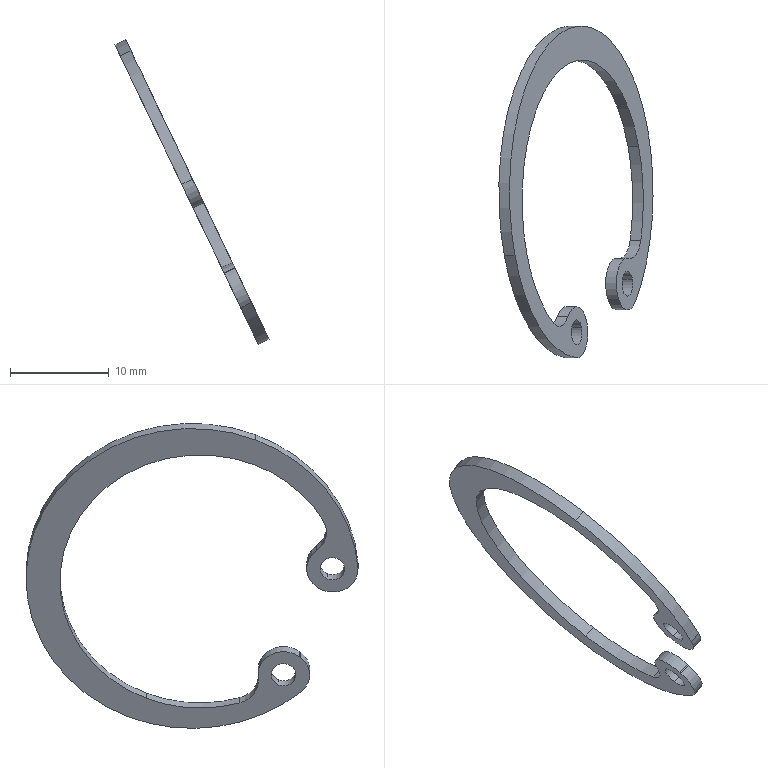Component | SolidWorks | AHTF30S5M100-1_RTWN32-1 | 1 solid | 21 faces | box 15.63 x 33.67 x 30.91 mm | volume 309 mm3 | cylinder 17 | plane 4 | commonest cylinder face diameters 5.2 x5 2.5 x4 28.45 x3 33.7 x3 5 x2
build123d program:
from build123d import *

# Parameters (mm, degrees)
BOSS_EXTRUDE1_DEPTH      = 0.6
BOSS_EXTRUDE1_DEPTH_BACK = 0.6
SKETCH1_R                = 1.25


with BuildPart() as part:
    # Sketch1 → Boss-Extrude1 (new, two sides: drawn at the far end of the back side and taken through both)
    with BuildSketch(Plane(origin=(0, 0, 0), x_dir=(0, 0, -1), z_dir=(1, 0, 0)).offset(-BOSS_EXTRUDE1_DEPTH_BACK)):
        with BuildLine():
            Line((-3.99, -13.556), (-3.956, -13.441))
            ThreePointArc((-3.956, -13.441), (-4.838, -10.667), (-7.741, -10.45))
            ThreePointArc((-7.741, -10.45), (-9.511, -10.749), (-11.053, -9.83))
            ThreePointArc((-11.053, -9.83), (0, 13.35), (11.053, -9.83))
            ThreePointArc((11.053, -9.83), (9.511, -10.749), (7.741, -10.45))
            ThreePointArc((7.741, -10.45), (4.838, -10.667), (3.956, -13.441))
            Line((3.956, -13.441), (3.99, -13.556))
            ThreePointArc((3.99, -13.556), (5.388, -15.141), (7.501, -15.088))
            ThreePointArc((7.501, -15.088), (0, 16.85), (-7.501, -15.088))
            ThreePointArc((-7.501, -15.088), (-5.388, -15.141), (-3.99, -13.556))
        make_face()
        with Locations((6.45, -12.707)):
            Circle(SKETCH1_R, mode=Mode.SUBTRACT)
        with Locations((-6.45, -12.707)):
            Circle(SKETCH1_R, mode=Mode.SUBTRACT)
    extrude(amount=BOSS_EXTRUDE1_DEPTH + BOSS_EXTRUDE1_DEPTH_BACK)


solid = part.part

# Placed as in the assembly
solid = solid.moved(Location((-5.543, 250, 455.725), (-155.302, 23.505, 169.606)))
STEP:
#1=COLOUR_RGB('',0.7922,0.8196,0.9333);
#2=FILL_AREA_STYLE_COLOUR('',#1);
#3=FILL_AREA_STYLE('',(#2));
#4=SURFACE_STYLE_FILL_AREA(#3);
#5=SURFACE_SIDE_STYLE('',(#4));
#6=SURFACE_STYLE_USAGE(.BOTH.,#5);
#7=PRESENTATION_STYLE_ASSIGNMENT((#6));
#8=CARTESIAN_POINT('',(-0.03588,9.497,17.506));
#9=VERTEX_POINT('',#8);
#10=CARTESIAN_POINT('',(-0.07514,9.459,17.588));
#11=VERTEX_POINT('',#10);
#12=CARTESIAN_POINT('',(-0.05551,9.478,17.547));
#13=DIRECTION('',(-0.902,0.,-0.4318));
#14=DIRECTION('',(-0.3988,-0.3832,0.8331));
#15=AXIS2_PLACEMENT_3D('',#12,#13,#14);
#16=CIRCLE('',#15,0.04921);
#17=EDGE_CURVE('',#9,#11,#16,.T.);
#18=ORIENTED_EDGE('',*,*,#17,.T.);
#19=CARTESIAN_POINT('',(-0.03252,9.459,17.609));
#20=VERTEX_POINT('',#19);
#21=CARTESIAN_POINT('',(-0.07514,9.459,17.588));
#22=DIRECTION('',(0.902,-0.,0.4318));
#23=VECTOR('',#22,39.37);
#24=LINE('',#21,#23);
#25=EDGE_CURVE('',#11,#20,#24,.T.);
#26=ORIENTED_EDGE('',*,*,#25,.T.);
#27=CARTESIAN_POINT('',(0.006732,9.497,17.527));
#28=VERTEX_POINT('',#27);
#29=CARTESIAN_POINT('',(-0.0129,9.478,17.568));
#30=DIRECTION('',(-0.902,0.,-0.4318));
#31=DIRECTION('',(-0.3988,-0.3832,0.8331));
#32=AXIS2_PLACEMENT_3D('',#29,#30,#31);
#33=CIRCLE('',#32,0.04921);
#34=EDGE_CURVE('',#28,#20,#33,.T.);
#35=ORIENTED_EDGE('',*,*,#34,.F.);
#36=CARTESIAN_POINT('',(-0.03588,9.497,17.506));
#37=DIRECTION('',(0.902,-0.,0.4318));
#38=VECTOR('',#37,39.37);
#39=LINE('',#36,#38);
#40=EDGE_CURVE('',#9,#28,#39,.T.);
#41=ORIENTED_EDGE('',*,*,#40,.F.);
#42=EDGE_LOOP('',(#18,#26,#35,#41));
#43=FACE_OUTER_BOUND('',#42,.T.);
#44=CARTESIAN_POINT('',(-0.05551,9.478,17.547));
#45=DIRECTION('',(0.902,-0.,0.4318));
#46=DIRECTION('',(0.3988,0.3832,-0.8331));
#47=AXIS2_PLACEMENT_3D('',#44,#45,#46);
#48=CYLINDRICAL_SURFACE('',#47,0.04921);
#49=ADVANCED_FACE('',(#43),#48,.F.);
#50=CARTESIAN_POINT('',(-0.2384,9.302,17.929));
#51=VERTEX_POINT('',#50);
#52=CARTESIAN_POINT('',(-0.2777,9.264,18.011));
#53=VERTEX_POINT('',#52);
#54=CARTESIAN_POINT('',(-0.2581,9.283,17.97));
#55=DIRECTION('',(-0.902,0.,-0.4318));
#56=DIRECTION('',(-0.3988,-0.3832,0.8331));
#57=AXIS2_PLACEMENT_3D('',#54,#55,#56);
#58=CIRCLE('',#57,0.04921);
#59=EDGE_CURVE('',#51,#53,#58,.T.);
#60=ORIENTED_EDGE('',*,*,#59,.T.);
#61=CARTESIAN_POINT('',(-0.2351,9.264,18.032));
#62=VERTEX_POINT('',#61);
#63=CARTESIAN_POINT('',(-0.2777,9.264,18.011));
#64=DIRECTION('',(0.902,-0.,0.4318));
#65=VECTOR('',#64,39.37);
#66=LINE('',#63,#65);
#67=EDGE_CURVE('',#53,#62,#66,.T.);
#68=ORIENTED_EDGE('',*,*,#67,.T.);
#69=CARTESIAN_POINT('',(-0.1958,9.302,17.95));
#70=VERTEX_POINT('',#69);
#71=CARTESIAN_POINT('',(-0.2155,9.283,17.991));
#72=DIRECTION('',(-0.902,0.,-0.4318));
#73=DIRECTION('',(-0.3988,-0.3832,0.8331));
#74=AXIS2_PLACEMENT_3D('',#71,#72,#73);
#75=CIRCLE('',#74,0.04921);
#76=EDGE_CURVE('',#70,#62,#75,.T.);
#77=ORIENTED_EDGE('',*,*,#76,.F.);
#78=CARTESIAN_POINT('',(-0.2384,9.302,17.929));
#79=DIRECTION('',(0.902,-0.,0.4318));
#80=VECTOR('',#79,39.37);
#81=LINE('',#78,#80);
#82=EDGE_CURVE('',#51,#70,#81,.T.);
#83=ORIENTED_EDGE('',*,*,#82,.F.);
#84=EDGE_LOOP('',(#60,#68,#77,#83));
#85=FACE_OUTER_BOUND('',#84,.T.);
#86=CARTESIAN_POINT('',(-0.2581,9.283,17.97));
#87=DIRECTION('',(0.902,-0.,0.4318));
#88=DIRECTION('',(0.3988,0.3832,-0.8331));
#89=AXIS2_PLACEMENT_3D('',#86,#87,#88);
#90=CYLINDRICAL_SURFACE('',#89,0.04921);
#91=ADVANCED_FACE('',(#85),#90,.F.);
#92=CARTESIAN_POINT('',(-0.2172,9.322,17.885));
#93=VERTEX_POINT('',#92);
#94=CARTESIAN_POINT('',(-0.2141,9.294,17.879));
#95=VERTEX_POINT('',#94);
#96=CARTESIAN_POINT('',(-0.2581,9.283,17.97));
#97=DIRECTION('',(-0.902,0.,-0.4318));
#98=DIRECTION('',(-0.3988,-0.3832,0.8331));
#99=AXIS2_PLACEMENT_3D('',#96,#97,#98);
#100=CIRCLE('',#99,0.1024);
#101=EDGE_CURVE('',#93,#95,#100,.T.);
#102=ORIENTED_EDGE('',*,*,#101,.F.);
#103=CARTESIAN_POINT('',(-0.1746,9.322,17.906));
#104=VERTEX_POINT('',#103);
#105=CARTESIAN_POINT('',(-0.2172,9.322,17.885));
#106=DIRECTION('',(0.902,-0.,0.4318));
#107=VECTOR('',#106,39.37);
#108=LINE('',#105,#107);
#109=EDGE_CURVE('',#93,#104,#108,.T.);
#110=ORIENTED_EDGE('',*,*,#109,.T.);
#111=CARTESIAN_POINT('',(-0.1715,9.294,17.899));
#112=VERTEX_POINT('',#111);
#113=CARTESIAN_POINT('',(-0.2155,9.283,17.991));
#114=DIRECTION('',(-0.902,0.,-0.4318));
#115=DIRECTION('',(-0.3988,-0.3832,0.8331));
#116=AXIS2_PLACEMENT_3D('',#113,#114,#115);
#117=CIRCLE('',#116,0.1024);
#118=EDGE_CURVE('',#104,#112,#117,.T.);
#119=ORIENTED_EDGE('',*,*,#118,.T.);
#120=CARTESIAN_POINT('',(-0.2141,9.294,17.879));
#121=DIRECTION('',(0.902,-0.,0.4318));
#122=VECTOR('',#121,39.37);
#123=LINE('',#120,#122);
#124=EDGE_CURVE('',#95,#112,#123,.T.);
#125=ORIENTED_EDGE('',*,*,#124,.F.);
#126=EDGE_LOOP('',(#102,#110,#119,#125));
#127=FACE_OUTER_BOUND('',#126,.T.);
#128=CARTESIAN_POINT('',(-0.2581,9.283,17.97));
#129=DIRECTION('',(0.902,-0.,0.4318));
#130=DIRECTION('',(0.3988,0.3832,-0.8331));
#131=AXIS2_PLACEMENT_3D('',#128,#129,#130);
#132=CYLINDRICAL_SURFACE('',#131,0.1024);
#133=ADVANCED_FACE('',(#127),#132,.T.);
#134=CARTESIAN_POINT('',(-0.4572,9.596,18.386));
#135=VERTEX_POINT('',#134);
#136=CARTESIAN_POINT('',(-0.3491,9.318,18.161));
#137=VERTEX_POINT('',#136);
#138=CARTESIAN_POINT('',(-0.2339,9.811,17.92));
#139=DIRECTION('',(0.902,-0.,0.4318));
#140=DIRECTION('',(0.3988,0.3832,-0.8331));
#141=AXIS2_PLACEMENT_3D('',#138,#139,#140);
#142=CIRCLE('',#141,0.56);
#143=EDGE_CURVE('',#135,#137,#142,.T.);
#144=ORIENTED_EDGE('',*,*,#143,.F.);
#145=CARTESIAN_POINT('',(-0.4146,9.596,18.407));
#146=VERTEX_POINT('',#145);
#147=CARTESIAN_POINT('',(-0.4572,9.596,18.386));
#148=DIRECTION('',(0.902,-0.,0.4318));
#149=VECTOR('',#148,39.37);
#150=LINE('',#147,#149);
#151=EDGE_CURVE('',#135,#146,#150,.T.);
#152=ORIENTED_EDGE('',*,*,#151,.T.);
#153=CARTESIAN_POINT('',(-0.3065,9.318,18.181));
#154=VERTEX_POINT('',#153);
#155=CARTESIAN_POINT('',(-0.1912,9.811,17.94));
#156=DIRECTION('',(0.902,-0.,0.4318));
#157=DIRECTION('',(0.3988,0.3832,-0.8331));
#158=AXIS2_PLACEMENT_3D('',#155,#156,#157);
#159=CIRCLE('',#158,0.56);
#160=EDGE_CURVE('',#146,#154,#159,.T.);
#161=ORIENTED_EDGE('',*,*,#160,.T.);
#162=CARTESIAN_POINT('',(-0.3491,9.318,18.161));
#163=DIRECTION('',(0.902,-0.,0.4318));
#164=VECTOR('',#163,39.37);
#165=LINE('',#162,#164);
#166=EDGE_CURVE('',#137,#154,#165,.T.);
#167=ORIENTED_EDGE('',*,*,#166,.F.);
#168=EDGE_LOOP('',(#144,#152,#161,#167));
#169=FACE_OUTER_BOUND('',#168,.T.);
#170=CARTESIAN_POINT('',(-0.2339,9.811,17.92));
#171=DIRECTION('',(0.902,-0.,0.4318));
#172=DIRECTION('',(0.3988,0.3832,-0.8331));
#173=AXIS2_PLACEMENT_3D('',#170,#171,#172);
#174=CYLINDRICAL_SURFACE('',#173,0.56);
#175=ADVANCED_FACE('',(#169),#174,.F.);
#176=ORIENTED_EDGE('',*,*,#151,.F.);
#177=CARTESIAN_POINT('',(-0.01049,10.025,17.453));
#178=VERTEX_POINT('',#177);
#179=CARTESIAN_POINT('',(-0.2339,9.811,17.92));
#180=DIRECTION('',(0.902,-0.,0.4318));
#181=DIRECTION('',(0.3988,0.3832,-0.8331));
#182=AXIS2_PLACEMENT_3D('',#179,#180,#181);
#183=CIRCLE('',#182,0.56);
#184=EDGE_CURVE('',#178,#135,#183,.T.);
#185=ORIENTED_EDGE('',*,*,#184,.F.);
#186=CARTESIAN_POINT('',(0.03212,10.025,17.474));
#187=VERTEX_POINT('',#186);
#188=CARTESIAN_POINT('',(-0.01049,10.025,17.453));
#189=DIRECTION('',(0.902,-0.,0.4318));
#190=VECTOR('',#189,39.37);
#191=LINE('',#188,#190);
#192=EDGE_CURVE('',#178,#187,#191,.T.);
#193=ORIENTED_EDGE('',*,*,#192,.T.);
#194=CARTESIAN_POINT('',(-0.1912,9.811,17.94));
#195=DIRECTION('',(0.902,-0.,0.4318));
#196=DIRECTION('',(0.3988,0.3832,-0.8331));
#197=AXIS2_PLACEMENT_3D('',#194,#195,#196);
#198=CIRCLE('',#197,0.56);
#199=EDGE_CURVE('',#187,#146,#198,.T.);
#200=ORIENTED_EDGE('',*,*,#199,.T.);
#201=EDGE_LOOP('',(#176,#185,#193,#200));
#202=FACE_OUTER_BOUND('',#201,.T.);
#203=CARTESIAN_POINT('',(-0.2339,9.811,17.92));
#204=DIRECTION('',(0.902,-0.,0.4318));
#205=DIRECTION('',(0.3988,0.3832,-0.8331));
#206=AXIS2_PLACEMENT_3D('',#203,#204,#205);
#207=CYLINDRICAL_SURFACE('',#206,0.56);
#208=ADVANCED_FACE('',(#202),#207,.F.);
#209=CARTESIAN_POINT('',(-0.5041,9.588,18.484));
#210=VERTEX_POINT('',#209);
#211=CARTESIAN_POINT('',(0.02503,10.097,17.379));
#212=VERTEX_POINT('',#211);
#213=CARTESIAN_POINT('',(-0.2396,9.843,17.932));
#214=DIRECTION('',(-0.902,0.,-0.4318));
#215=DIRECTION('',(-0.3988,-0.3832,0.8331));
#216=AXIS2_PLACEMENT_3D('',#213,#214,#215);
#217=CIRCLE('',#216,0.6634);
#218=EDGE_CURVE('',#210,#212,#217,.T.);
#219=ORIENTED_EDGE('',*,*,#218,.F.);
#220=CARTESIAN_POINT('',(-0.4615,9.588,18.505));
#221=VERTEX_POINT('',#220);
#222=CARTESIAN_POINT('',(-0.5041,9.588,18.484));
#223=DIRECTION('',(0.902,-0.,0.4318));
#224=VECTOR('',#223,39.37);
#225=LINE('',#222,#224);
#226=EDGE_CURVE('',#210,#221,#225,.T.);
#227=ORIENTED_EDGE('',*,*,#226,.T.);
#228=CARTESIAN_POINT('',(0.06764,10.097,17.399));
#229=VERTEX_POINT('',#228);
#230=CARTESIAN_POINT('',(-0.1969,9.843,17.952));
#231=DIRECTION('',(-0.902,0.,-0.4318));
#232=DIRECTION('',(-0.3988,-0.3832,0.8331));
#233=AXIS2_PLACEMENT_3D('',#230,#231,#232);
#234=CIRCLE('',#233,0.6634);
#235=EDGE_CURVE('',#221,#229,#234,.T.);
#236=ORIENTED_EDGE('',*,*,#235,.T.);
#237=CARTESIAN_POINT('',(0.02503,10.097,17.379));
#238=DIRECTION('',(0.902,-0.,0.4318));
#239=VECTOR('',#238,39.37);
#240=LINE('',#237,#239);
#241=EDGE_CURVE('',#212,#229,#240,.T.);
#242=ORIENTED_EDGE('',*,*,#241,.F.);
#243=EDGE_LOOP('',(#219,#227,#236,#242));
#244=FACE_OUTER_BOUND('',#243,.T.);
#245=CARTESIAN_POINT('',(-0.2396,9.843,17.932));
#246=DIRECTION('',(0.902,-0.,0.4318));
#247=DIRECTION('',(0.3988,0.3832,-0.8331));
#248=AXIS2_PLACEMENT_3D('',#245,#246,#247);
#249=CYLINDRICAL_SURFACE('',#248,0.6634);
#250=ADVANCED_FACE('',(#244),#249,.T.);
#251=CARTESIAN_POINT('',(-0.0235,9.407,17.48));
#252=VERTEX_POINT('',#251);
#253=CARTESIAN_POINT('',(-0.2396,9.843,17.932));
#254=DIRECTION('',(-0.902,0.,-0.4318));
#255=DIRECTION('',(-0.3988,-0.3832,0.8331));
#256=AXIS2_PLACEMENT_3D('',#253,#254,#255);
#257=CIRCLE('',#256,0.6634);
#258=EDGE_CURVE('',#212,#252,#257,.T.);
#259=ORIENTED_EDGE('',*,*,#258,.F.);
#260=ORIENTED_EDGE('',*,*,#241,.T.);
#261=CARTESIAN_POINT('',(0.01912,9.407,17.501));
#262=VERTEX_POINT('',#261);
#263=CARTESIAN_POINT('',(-0.1969,9.843,17.952));
#264=DIRECTION('',(-0.902,0.,-0.4318));
#265=DIRECTION('',(-0.3988,-0.3832,0.8331));
#266=AXIS2_PLACEMENT_3D('',#263,#264,#265);
#267=CIRCLE('',#266,0.6634);
#268=EDGE_CURVE('',#229,#262,#267,.T.);
#269=ORIENTED_EDGE('',*,*,#268,.T.);
#270=CARTESIAN_POINT('',(-0.0235,9.407,17.48));
#271=DIRECTION('',(0.902,-0.,0.4318));
#272=VECTOR('',#271,39.37);
#273=LINE('',#270,#272);
#274=EDGE_CURVE('',#252,#262,#273,.T.);
#275=ORIENTED_EDGE('',*,*,#274,.F.);
#276=EDGE_LOOP('',(#259,#260,#269,#275));
#277=FACE_OUTER_BOUND('',#276,.T.);
#278=CARTESIAN_POINT('',(-0.2396,9.843,17.932));
#279=DIRECTION('',(0.902,-0.,0.4318));
#280=DIRECTION('',(0.3988,0.3832,-0.8331));
#281=AXIS2_PLACEMENT_3D('',#278,#279,#280);
#282=CYLINDRICAL_SURFACE('',#281,0.6634);
#283=ADVANCED_FACE('',(#277),#282,.T.);
#284=ORIENTED_EDGE('',*,*,#59,.F.);
#285=CARTESIAN_POINT('',(-0.2581,9.283,17.97));
#286=DIRECTION('',(-0.902,0.,-0.4318));
#287=DIRECTION('',(-0.3988,-0.3832,0.8331));
#288=AXIS2_PLACEMENT_3D('',#285,#286,#287);
#289=CIRCLE('',#288,0.04921);
#290=EDGE_CURVE('',#53,#51,#289,.T.);
#291=ORIENTED_EDGE('',*,*,#290,.F.);
#292=EDGE_LOOP('',(#284,#291));
#293=FACE_BOUND('',#292,.T.);
#294=CARTESIAN_POINT('',(-0.2139,9.289,17.878));
#295=VERTEX_POINT('',#294);
#296=CARTESIAN_POINT('',(-0.259,9.181,17.972));
#297=VERTEX_POINT('',#296);
#298=CARTESIAN_POINT('',(-0.2562,9.279,17.966));
#299=DIRECTION('',(-0.902,0.,-0.4318));
#300=DIRECTION('',(-0.3988,-0.3832,0.8331));
#301=AXIS2_PLACEMENT_3D('',#298,#299,#300);
#302=CIRCLE('',#301,0.09843);
#303=EDGE_CURVE('',#295,#297,#302,.T.);
#304=ORIENTED_EDGE('',*,*,#303,.T.);
#305=CARTESIAN_POINT('',(-0.2396,9.843,17.932));
#306=DIRECTION('',(-0.902,0.,-0.4318));
#307=DIRECTION('',(-0.3988,-0.3832,0.8331));
#308=AXIS2_PLACEMENT_3D('',#305,#306,#307);
#309=CIRCLE('',#308,0.6634);
#310=EDGE_CURVE('',#297,#210,#309,.T.);
#311=ORIENTED_EDGE('',*,*,#310,.T.);
#312=ORIENTED_EDGE('',*,*,#218,.T.);
#313=ORIENTED_EDGE('',*,*,#258,.T.);
#314=CARTESIAN_POINT('',(-0.08861,9.41,17.616));
#315=VERTEX_POINT('',#314);
#316=CARTESIAN_POINT('',(-0.05555,9.472,17.547));
#317=DIRECTION('',(-0.902,0.,-0.4318));
#318=DIRECTION('',(-0.3988,-0.3832,0.8331));
#319=AXIS2_PLACEMENT_3D('',#316,#317,#318);
#320=CIRCLE('',#319,0.09843);
#321=EDGE_CURVE('',#252,#315,#320,.T.);
#322=ORIENTED_EDGE('',*,*,#321,.T.);
#323=CARTESIAN_POINT('',(-0.08989,9.413,17.619));
#324=VERTEX_POINT('',#323);
#325=CARTESIAN_POINT('',(-0.08861,9.41,17.616));
#326=DIRECTION('',(-0.2713,0.7779,0.5668));
#327=VECTOR('',#326,39.37);
#328=LINE('',#325,#327);
#329=EDGE_CURVE('',#315,#324,#328,.T.);
#330=ORIENTED_EDGE('',*,*,#329,.T.);
#331=CARTESIAN_POINT('',(-0.04993,9.579,17.536));
#332=VERTEX_POINT('',#331);
#333=CARTESIAN_POINT('',(-0.05551,9.478,17.547));
#334=DIRECTION('',(-0.902,0.,-0.4318));
#335=DIRECTION('',(-0.3988,-0.3832,0.8331));
#336=AXIS2_PLACEMENT_3D('',#333,#334,#335);
#337=CIRCLE('',#336,0.1024);
#338=EDGE_CURVE('',#324,#332,#337,.T.);
#339=ORIENTED_EDGE('',*,*,#338,.T.);
#340=CARTESIAN_POINT('',(-0.001977,9.652,17.435));
#341=VERTEX_POINT('',#340);
#342=CARTESIAN_POINT('',(-0.04436,9.681,17.524));
#343=DIRECTION('',(0.902,-0.,0.4318));
#344=DIRECTION('',(0.3988,0.3832,-0.8331));
#345=AXIS2_PLACEMENT_3D('',#342,#343,#344);
#346=CIRCLE('',#345,0.1024);
#347=EDGE_CURVE('',#332,#341,#346,.T.);
#348=ORIENTED_EDGE('',*,*,#347,.T.);
#349=CARTESIAN_POINT('',(-0.2339,9.811,17.92));
#350=DIRECTION('',(0.902,-0.,0.4318));
#351=DIRECTION('',(0.3988,0.3832,-0.8331));
#352=AXIS2_PLACEMENT_3D('',#349,#350,#351);
#353=CIRCLE('',#352,0.56);
#354=EDGE_CURVE('',#341,#178,#353,.T.);
#355=ORIENTED_EDGE('',*,*,#354,.T.);
#356=ORIENTED_EDGE('',*,*,#184,.T.);
#357=ORIENTED_EDGE('',*,*,#143,.T.);
#358=CARTESIAN_POINT('',(-0.293,9.346,18.043));
#359=VERTEX_POINT('',#358);
#360=CARTESIAN_POINT('',(-0.328,9.408,18.117));
#361=DIRECTION('',(0.902,-0.,0.4318));
#362=DIRECTION('',(0.3988,0.3832,-0.8331));
#363=AXIS2_PLACEMENT_3D('',#360,#361,#362);
#364=CIRCLE('',#363,0.1024);
#365=EDGE_CURVE('',#137,#359,#364,.T.);
#366=ORIENTED_EDGE('',*,*,#365,.T.);
#367=CARTESIAN_POINT('',(-0.2581,9.283,17.97));
#368=DIRECTION('',(-0.902,0.,-0.4318));
#369=DIRECTION('',(-0.3988,-0.3832,0.8331));
#370=AXIS2_PLACEMENT_3D('',#367,#368,#369);
#371=CIRCLE('',#370,0.1024);
#372=EDGE_CURVE('',#359,#93,#371,.T.);
#373=ORIENTED_EDGE('',*,*,#372,.T.);
#374=ORIENTED_EDGE('',*,*,#101,.T.);
#375=CARTESIAN_POINT('',(-0.2141,9.294,17.879));
#376=DIRECTION('',(0.04611,-0.9943,-0.09632));
#377=VECTOR('',#376,39.37);
#378=LINE('',#375,#377);
#379=EDGE_CURVE('',#95,#295,#378,.T.);
#380=ORIENTED_EDGE('',*,*,#379,.T.);
#381=EDGE_LOOP('',(#304,#311,#312,#313,#322,#330,#339,#348,#355,#356,#357,#366,#373,#374,#380));
#382=FACE_OUTER_BOUND('',#381,.T.);
#383=ORIENTED_EDGE('',*,*,#17,.F.);
#384=CARTESIAN_POINT('',(-0.05551,9.478,17.547));
#385=DIRECTION('',(-0.902,0.,-0.4318));
#386=DIRECTION('',(-0.3988,-0.3832,0.8331));
#387=AXIS2_PLACEMENT_3D('',#384,#385,#386);
#388=CIRCLE('',#387,0.04921);
#389=EDGE_CURVE('',#11,#9,#388,.T.);
#390=ORIENTED_EDGE('',*,*,#389,.F.);
#391=EDGE_LOOP('',(#383,#390));
#392=FACE_BOUND('',#391,.T.);
#393=CARTESIAN_POINT('',(-0.2562,9.279,17.966));
#394=DIRECTION('',(-0.902,0.,-0.4318));
#395=DIRECTION('',(-0.3988,-0.3832,0.8331));
#396=AXIS2_PLACEMENT_3D('',#393,#394,#395);
#397=PLANE('',#396);
#398=ADVANCED_FACE('',(#293,#382,#392),#397,.T.);
#399=CARTESIAN_POINT('',(-0.1713,9.289,17.899));
#400=VERTEX_POINT('',#399);
#401=CARTESIAN_POINT('',(-0.2139,9.289,17.878));
#402=DIRECTION('',(0.902,-0.,0.4318));
#403=VECTOR('',#402,39.37);
#404=LINE('',#401,#403);
#405=EDGE_CURVE('',#295,#400,#404,.T.);
#406=ORIENTED_EDGE('',*,*,#405,.T.);
#407=CARTESIAN_POINT('',(-0.2164,9.181,17.993));
#408=VERTEX_POINT('',#407);
#409=CARTESIAN_POINT('',(-0.2135,9.279,17.987));
#410=DIRECTION('',(-0.902,0.,-0.4318));
#411=DIRECTION('',(-0.3988,-0.3832,0.8331));
#412=AXIS2_PLACEMENT_3D('',#409,#410,#411);
#413=CIRCLE('',#412,0.09843);
#414=EDGE_CURVE('',#400,#408,#413,.T.);
#415=ORIENTED_EDGE('',*,*,#414,.T.);
#416=CARTESIAN_POINT('',(-0.259,9.181,17.972));
#417=DIRECTION('',(0.902,-0.,0.4318));
#418=VECTOR('',#417,39.37);
#419=LINE('',#416,#418);
#420=EDGE_CURVE('',#297,#408,#419,.T.);
#421=ORIENTED_EDGE('',*,*,#420,.F.);
#422=ORIENTED_EDGE('',*,*,#303,.F.);
#423=EDGE_LOOP('',(#406,#415,#421,#422));
#424=FACE_OUTER_BOUND('',#423,.T.);
#425=CARTESIAN_POINT('',(-0.2562,9.279,17.966));
#426=DIRECTION('',(0.902,-0.,0.4318));
#427=DIRECTION('',(0.3988,0.3832,-0.8331));
#428=AXIS2_PLACEMENT_3D('',#425,#426,#427);
#429=CYLINDRICAL_SURFACE('',#428,0.09843);
#430=ADVANCED_FACE('',(#424),#429,.T.);
#431=ORIENTED_EDGE('',*,*,#226,.F.);
#432=ORIENTED_EDGE('',*,*,#310,.F.);
#433=ORIENTED_EDGE('',*,*,#420,.T.);
#434=CARTESIAN_POINT('',(-0.1969,9.843,17.952));
#435=DIRECTION('',(-0.902,0.,-0.4318));
#436=DIRECTION('',(-0.3988,-0.3832,0.8331));
#437=AXIS2_PLACEMENT_3D('',#434,#435,#436);
#438=CIRCLE('',#437,0.6634);
#439=EDGE_CURVE('',#408,#221,#438,.T.);
#440=ORIENTED_EDGE('',*,*,#439,.T.);
#441=EDGE_LOOP('',(#431,#432,#433,#440));
#442=FACE_OUTER_BOUND('',#441,.T.);
#443=CARTESIAN_POINT('',(-0.2396,9.843,17.932));
#444=DIRECTION('',(0.902,-0.,0.4318));
#445=DIRECTION('',(0.3988,0.3832,-0.8331));
#446=AXIS2_PLACEMENT_3D('',#443,#444,#445);
#447=CYLINDRICAL_SURFACE('',#446,0.6634);
#448=ADVANCED_FACE('',(#442),#447,.T.);
#449=ORIENTED_EDGE('',*,*,#274,.T.);
#450=CARTESIAN_POINT('',(-0.046,9.41,17.637));
#451=VERTEX_POINT('',#450);
#452=CARTESIAN_POINT('',(-0.01294,9.472,17.568));
#453=DIRECTION('',(-0.902,0.,-0.4318));
#454=DIRECTION('',(-0.3988,-0.3832,0.8331));
#455=AXIS2_PLACEMENT_3D('',#452,#453,#454);
#456=CIRCLE('',#455,0.09843);
#457=EDGE_CURVE('',#262,#451,#456,.T.);
#458=ORIENTED_EDGE('',*,*,#457,.T.);
#459=CARTESIAN_POINT('',(-0.08861,9.41,17.616));
#460=DIRECTION('',(0.902,-0.,0.4318));
#461=VECTOR('',#460,39.37);
#462=LINE('',#459,#461);
#463=EDGE_CURVE('',#315,#451,#462,.T.);
#464=ORIENTED_EDGE('',*,*,#463,.F.);
#465=ORIENTED_EDGE('',*,*,#321,.F.);
#466=EDGE_LOOP('',(#449,#458,#464,#465));
#467=FACE_OUTER_BOUND('',#466,.T.);
#468=CARTESIAN_POINT('',(-0.05555,9.472,17.547));
#469=DIRECTION('',(0.902,-0.,0.4318));
#470=DIRECTION('',(0.3988,0.3832,-0.8331));
#471=AXIS2_PLACEMENT_3D('',#468,#469,#470);
#472=CYLINDRICAL_SURFACE('',#471,0.09843);
#473=ADVANCED_FACE('',(#467),#472,.T.);
#474=ORIENTED_EDGE('',*,*,#463,.T.);
#475=CARTESIAN_POINT('',(-0.04728,9.413,17.639));
#476=VERTEX_POINT('',#475);
#477=CARTESIAN_POINT('',(-0.046,9.41,17.637));
#478=DIRECTION('',(-0.2713,0.7779,0.5668));
#479=VECTOR('',#478,39.37);
#480=LINE('',#477,#479);
#481=EDGE_CURVE('',#451,#476,#480,.T.);
#482=ORIENTED_EDGE('',*,*,#481,.T.);
#483=CARTESIAN_POINT('',(-0.08989,9.413,17.619));
#484=DIRECTION('',(0.902,-0.,0.4318));
#485=VECTOR('',#484,39.37);
#486=LINE('',#483,#485);
#487=EDGE_CURVE('',#324,#476,#486,.T.);
#488=ORIENTED_EDGE('',*,*,#487,.F.);
#489=ORIENTED_EDGE('',*,*,#329,.F.);
#490=EDGE_LOOP('',(#474,#482,#488,#489));
#491=FACE_OUTER_BOUND('',#490,.T.);
#492=CARTESIAN_POINT('',(-0.08861,9.41,17.616));
#493=DIRECTION('',(0.3359,0.6284,-0.7017));
#494=DIRECTION('',(0.2713,-0.7779,-0.5668));
#495=AXIS2_PLACEMENT_3D('',#492,#493,#494);
#496=PLANE('',#495);
#497=ADVANCED_FACE('',(#491),#496,.F.);
#498=ORIENTED_EDGE('',*,*,#487,.T.);
#499=CARTESIAN_POINT('',(-0.00732,9.579,17.556));
#500=VERTEX_POINT('',#499);
#501=CARTESIAN_POINT('',(-0.0129,9.478,17.568));
#502=DIRECTION('',(-0.902,0.,-0.4318));
#503=DIRECTION('',(-0.3988,-0.3832,0.8331));
#504=AXIS2_PLACEMENT_3D('',#501,#502,#503);
#505=CIRCLE('',#504,0.1024);
#506=EDGE_CURVE('',#476,#500,#505,.T.);
#507=ORIENTED_EDGE('',*,*,#506,.T.);
#508=CARTESIAN_POINT('',(-0.04993,9.579,17.536));
#509=DIRECTION('',(0.902,-0.,0.4318));
#510=VECTOR('',#509,39.37);
#511=LINE('',#508,#510);
#512=EDGE_CURVE('',#332,#500,#511,.T.);
#513=ORIENTED_EDGE('',*,*,#512,.F.);
#514=ORIENTED_EDGE('',*,*,#338,.F.);
#515=EDGE_LOOP('',(#498,#507,#513,#514));
#516=FACE_OUTER_BOUND('',#515,.T.);
#517=CARTESIAN_POINT('',(-0.05551,9.478,17.547));
#518=DIRECTION('',(0.902,-0.,0.4318));
#519=DIRECTION('',(0.3988,0.3832,-0.8331));
#520=AXIS2_PLACEMENT_3D('',#517,#518,#519);
#521=CYLINDRICAL_SURFACE('',#520,0.1024);
#522=ADVANCED_FACE('',(#516),#521,.T.);
#523=ORIENTED_EDGE('',*,*,#512,.T.);
#524=CARTESIAN_POINT('',(0.04064,9.652,17.456));
#525=VERTEX_POINT('',#524);
#526=CARTESIAN_POINT('',(-0.001745,9.681,17.544));
#527=DIRECTION('',(0.902,-0.,0.4318));
#528=DIRECTION('',(0.3988,0.3832,-0.8331));
#529=AXIS2_PLACEMENT_3D('',#526,#527,#528);
#530=CIRCLE('',#529,0.1024);
#531=EDGE_CURVE('',#500,#525,#530,.T.);
#532=ORIENTED_EDGE('',*,*,#531,.T.);
#533=CARTESIAN_POINT('',(-0.001977,9.652,17.435));
#534=DIRECTION('',(0.902,-0.,0.4318));
#535=VECTOR('',#534,39.37);
#536=LINE('',#533,#535);
#537=EDGE_CURVE('',#341,#525,#536,.T.);
#538=ORIENTED_EDGE('',*,*,#537,.F.);
#539=ORIENTED_EDGE('',*,*,#347,.F.);
#540=EDGE_LOOP('',(#523,#532,#538,#539));
#541=FACE_OUTER_BOUND('',#540,.T.);
#542=CARTESIAN_POINT('',(-0.04436,9.681,17.524));
#543=DIRECTION('',(0.902,-0.,0.4318));
#544=DIRECTION('',(0.3988,0.3832,-0.8331));
#545=AXIS2_PLACEMENT_3D('',#542,#543,#544);
#546=CYLINDRICAL_SURFACE('',#545,0.1024);
#547=ADVANCED_FACE('',(#541),#546,.F.);
#548=ORIENTED_EDGE('',*,*,#192,.F.);
#549=ORIENTED_EDGE('',*,*,#354,.F.);
#550=ORIENTED_EDGE('',*,*,#537,.T.);
#551=CARTESIAN_POINT('',(-0.1912,9.811,17.94));
#552=DIRECTION('',(0.902,-0.,0.4318));
#553=DIRECTION('',(0.3988,0.3832,-0.8331));
#554=AXIS2_PLACEMENT_3D('',#551,#552,#553);
#555=CIRCLE('',#554,0.56);
#556=EDGE_CURVE('',#525,#187,#555,.T.);
#557=ORIENTED_EDGE('',*,*,#556,.T.);
#558=EDGE_LOOP('',(#548,#549,#550,#557));
#559=FACE_OUTER_BOUND('',#558,.T.);
#560=CARTESIAN_POINT('',(-0.2339,9.811,17.92));
#561=DIRECTION('',(0.902,-0.,0.4318));
#562=DIRECTION('',(0.3988,0.3832,-0.8331));
#563=AXIS2_PLACEMENT_3D('',#560,#561,#562);
#564=CYLINDRICAL_SURFACE('',#563,0.56);
#565=ADVANCED_FACE('',(#559),#564,.F.);
#566=ORIENTED_EDGE('',*,*,#166,.T.);
#567=CARTESIAN_POINT('',(-0.2504,9.346,18.064));
#568=VERTEX_POINT('',#567);
#569=CARTESIAN_POINT('',(-0.2854,9.408,18.137));
#570=DIRECTION('',(0.902,-0.,0.4318));
#571=DIRECTION('',(0.3988,0.3832,-0.8331));
#572=AXIS2_PLACEMENT_3D('',#569,#570,#571);
#573=CIRCLE('',#572,0.1024);
#574=EDGE_CURVE('',#154,#568,#573,.T.);
#575=ORIENTED_EDGE('',*,*,#574,.T.);
#576=CARTESIAN_POINT('',(-0.293,9.346,18.043));
#577=DIRECTION('',(0.902,-0.,0.4318));
#578=VECTOR('',#577,39.37);
#579=LINE('',#576,#578);
#580=EDGE_CURVE('',#359,#568,#579,.T.);
#581=ORIENTED_EDGE('',*,*,#580,.F.);
#582=ORIENTED_EDGE('',*,*,#365,.F.);
#583=EDGE_LOOP('',(#566,#575,#581,#582));
#584=FACE_OUTER_BOUND('',#583,.T.);
#585=CARTESIAN_POINT('',(-0.328,9.408,18.117));
#586=DIRECTION('',(0.902,-0.,0.4318));
#587=DIRECTION('',(0.3988,0.3832,-0.8331));
#588=AXIS2_PLACEMENT_3D('',#585,#586,#587);
#589=CYLINDRICAL_SURFACE('',#588,0.1024);
#590=ADVANCED_FACE('',(#584),#589,.F.);
#591=ORIENTED_EDGE('',*,*,#109,.F.);
#592=ORIENTED_EDGE('',*,*,#372,.F.);
#593=ORIENTED_EDGE('',*,*,#580,.T.);
#594=CARTESIAN_POINT('',(-0.2155,9.283,17.991));
#595=DIRECTION('',(-0.902,0.,-0.4318));
#596=DIRECTION('',(-0.3988,-0.3832,0.8331));
#597=AXIS2_PLACEMENT_3D('',#594,#595,#596);
#598=CIRCLE('',#597,0.1024);
#599=EDGE_CURVE('',#568,#104,#598,.T.);
#600=ORIENTED_EDGE('',*,*,#599,.T.);
#601=EDGE_LOOP('',(#591,#592,#593,#600));
#602=FACE_OUTER_BOUND('',#601,.T.);
#603=CARTESIAN_POINT('',(-0.2581,9.283,17.97));
#604=DIRECTION('',(0.902,-0.,0.4318));
#605=DIRECTION('',(0.3988,0.3832,-0.8331));
#606=AXIS2_PLACEMENT_3D('',#603,#604,#605);
#607=CYLINDRICAL_SURFACE('',#606,0.1024);
#608=ADVANCED_FACE('',(#602),#607,.T.);
#609=ORIENTED_EDGE('',*,*,#124,.T.);
#610=CARTESIAN_POINT('',(-0.1715,9.294,17.899));
#611=DIRECTION('',(0.04611,-0.9943,-0.09632));
#612=VECTOR('',#611,39.37);
#613=LINE('',#610,#612);
#614=EDGE_CURVE('',#112,#400,#613,.T.);
#615=ORIENTED_EDGE('',*,*,#614,.T.);
#616=ORIENTED_EDGE('',*,*,#405,.F.);
#617=ORIENTED_EDGE('',*,*,#379,.F.);
#618=EDGE_LOOP('',(#609,#615,#616,#617));
#619=FACE_OUTER_BOUND('',#618,.T.);
#620=CARTESIAN_POINT('',(-0.2141,9.294,17.879));
#621=DIRECTION('',(-0.4293,-0.1068,0.8968));
#622=DIRECTION('',(-0.04611,0.9943,0.09632));
#623=AXIS2_PLACEMENT_3D('',#620,#621,#622);
#624=PLANE('',#623);
#625=ADVANCED_FACE('',(#619),#624,.F.);
#626=ORIENTED_EDGE('',*,*,#67,.F.);
#627=ORIENTED_EDGE('',*,*,#290,.T.);
#628=ORIENTED_EDGE('',*,*,#82,.T.);
#629=CARTESIAN_POINT('',(-0.2155,9.283,17.991));
#630=DIRECTION('',(-0.902,0.,-0.4318));
#631=DIRECTION('',(-0.3988,-0.3832,0.8331));
#632=AXIS2_PLACEMENT_3D('',#629,#630,#631);
#633=CIRCLE('',#632,0.04921);
#634=EDGE_CURVE('',#62,#70,#633,.T.);
#635=ORIENTED_EDGE('',*,*,#634,.F.);
#636=EDGE_LOOP('',(#626,#627,#628,#635));
#637=FACE_OUTER_BOUND('',#636,.T.);
#638=CARTESIAN_POINT('',(-0.2581,9.283,17.97));
#639=DIRECTION('',(0.902,-0.,0.4318));
#640=DIRECTION('',(0.3988,0.3832,-0.8331));
#641=AXIS2_PLACEMENT_3D('',#638,#639,#640);
#642=CYLINDRICAL_SURFACE('',#641,0.04921);
#643=ADVANCED_FACE('',(#637),#642,.F.);
#644=ORIENTED_EDGE('',*,*,#25,.F.);
#645=ORIENTED_EDGE('',*,*,#389,.T.);
#646=ORIENTED_EDGE('',*,*,#40,.T.);
#647=CARTESIAN_POINT('',(-0.0129,9.478,17.568));
#648=DIRECTION('',(-0.902,0.,-0.4318));
#649=DIRECTION('',(-0.3988,-0.3832,0.8331));
#650=AXIS2_PLACEMENT_3D('',#647,#648,#649);
#651=CIRCLE('',#650,0.04921);
#652=EDGE_CURVE('',#20,#28,#651,.T.);
#653=ORIENTED_EDGE('',*,*,#652,.F.);
#654=EDGE_LOOP('',(#644,#645,#646,#653));
#655=FACE_OUTER_BOUND('',#654,.T.);
#656=CARTESIAN_POINT('',(-0.05551,9.478,17.547));
#657=DIRECTION('',(0.902,-0.,0.4318));
#658=DIRECTION('',(0.3988,0.3832,-0.8331));
#659=AXIS2_PLACEMENT_3D('',#656,#657,#658);
#660=CYLINDRICAL_SURFACE('',#659,0.04921);
#661=ADVANCED_FACE('',(#655),#660,.F.);
#662=ORIENTED_EDGE('',*,*,#34,.T.);
#663=ORIENTED_EDGE('',*,*,#652,.T.);
#664=EDGE_LOOP('',(#662,#663));
#665=FACE_BOUND('',#664,.T.);
#666=ORIENTED_EDGE('',*,*,#76,.T.);
#667=ORIENTED_EDGE('',*,*,#634,.T.);
#668=EDGE_LOOP('',(#666,#667));
#669=FACE_BOUND('',#668,.T.);
#670=ORIENTED_EDGE('',*,*,#414,.F.);
#671=ORIENTED_EDGE('',*,*,#614,.F.);
#672=ORIENTED_EDGE('',*,*,#118,.F.);
#673=ORIENTED_EDGE('',*,*,#599,.F.);
#674=ORIENTED_EDGE('',*,*,#574,.F.);
#675=ORIENTED_EDGE('',*,*,#160,.F.);
#676=ORIENTED_EDGE('',*,*,#199,.F.);
#677=ORIENTED_EDGE('',*,*,#556,.F.);
#678=ORIENTED_EDGE('',*,*,#531,.F.);
#679=ORIENTED_EDGE('',*,*,#506,.F.);
#680=ORIENTED_EDGE('',*,*,#481,.F.);
#681=ORIENTED_EDGE('',*,*,#457,.F.);
#682=ORIENTED_EDGE('',*,*,#268,.F.);
#683=ORIENTED_EDGE('',*,*,#235,.F.);
#684=ORIENTED_EDGE('',*,*,#439,.F.);
#685=EDGE_LOOP('',(#670,#671,#672,#673,#674,#675,#676,#677,#678,#679,#680,#681,#682,#683,#684));
#686=FACE_OUTER_BOUND('',#685,.T.);
#687=CARTESIAN_POINT('',(-0.2135,9.279,17.987));
#688=DIRECTION('',(-0.902,0.,-0.4318));
#689=DIRECTION('',(-0.3988,-0.3832,0.8331));
#690=AXIS2_PLACEMENT_3D('',#687,#688,#689);
#691=PLANE('',#690);
#692=ADVANCED_FACE('',(#665,#669,#686),#691,.F.);
#693=CLOSED_SHELL('',(#49,#91,#133,#175,#208,#250,#283,#398,#430,#448,#473,#497,#522,#547,#565,#590,#608,#625,#643,#661,#692));
#694=MANIFOLD_SOLID_BREP('',#693);
#695=STYLED_ITEM('',(#7),#694);
#696=(LENGTH_UNIT()NAMED_UNIT(*)SI_UNIT($,.METRE.));
#697=LENGTH_MEASURE_WITH_UNIT(LENGTH_MEASURE(0.0254),#696);
#698=DIMENSIONAL_EXPONENTS(1.,0.,0.,0.,0.,0.,0.);
#699=(CONVERSION_BASED_UNIT('',#697)LENGTH_UNIT()NAMED_UNIT(#698));
#700=UNCERTAINTY_MEASURE_WITH_UNIT(LENGTH_MEASURE(0.00001),#699,'','');
#701=(NAMED_UNIT(*)PLANE_ANGLE_UNIT()SI_UNIT($,.RADIAN.));
#702=(NAMED_UNIT(*)SI_UNIT($,.STERADIAN.)SOLID_ANGLE_UNIT());
#703=(GEOMETRIC_REPRESENTATION_CONTEXT(3)GLOBAL_UNCERTAINTY_ASSIGNED_CONTEXT((#700))GLOBAL_UNIT_ASSIGNED_CONTEXT((#699,#701,#702))REPRESENTATION_CONTEXT('',''));
#704=MECHANICAL_DESIGN_GEOMETRIC_PRESENTATION_REPRESENTATION('',(#695),#703);
#705=PRESENTATION_LAYER_ASSIGNMENT('','',(#695));
#706=CARTESIAN_POINT('',(0.,0.,0.));
#707=DIRECTION('',(0.,0.,1.));
#708=DIRECTION('',(1.,0.,0.));
#709=AXIS2_PLACEMENT_3D('',#706,#707,#708);
#710=(LENGTH_UNIT()NAMED_UNIT(*)SI_UNIT($,.METRE.));
#711=LENGTH_MEASURE_WITH_UNIT(LENGTH_MEASURE(0.0254),#710);
#712=DIMENSIONAL_EXPONENTS(1.,0.,0.,0.,0.,0.,0.);
#713=(CONVERSION_BASED_UNIT('',#711)LENGTH_UNIT()NAMED_UNIT(#712));
#714=UNCERTAINTY_MEASURE_WITH_UNIT(LENGTH_MEASURE(0.00001),#713,'','');
#715=(NAMED_UNIT(*)PLANE_ANGLE_UNIT()SI_UNIT($,.RADIAN.));
#716=(NAMED_UNIT(*)SI_UNIT($,.STERADIAN.)SOLID_ANGLE_UNIT());
#717=(GEOMETRIC_REPRESENTATION_CONTEXT(3)GLOBAL_UNCERTAINTY_ASSIGNED_CONTEXT((#714))GLOBAL_UNIT_ASSIGNED_CONTEXT((#713,#715,#716))REPRESENTATION_CONTEXT('',''));
#718=ADVANCED_BREP_SHAPE_REPRESENTATION('',(#694,#709),#717);